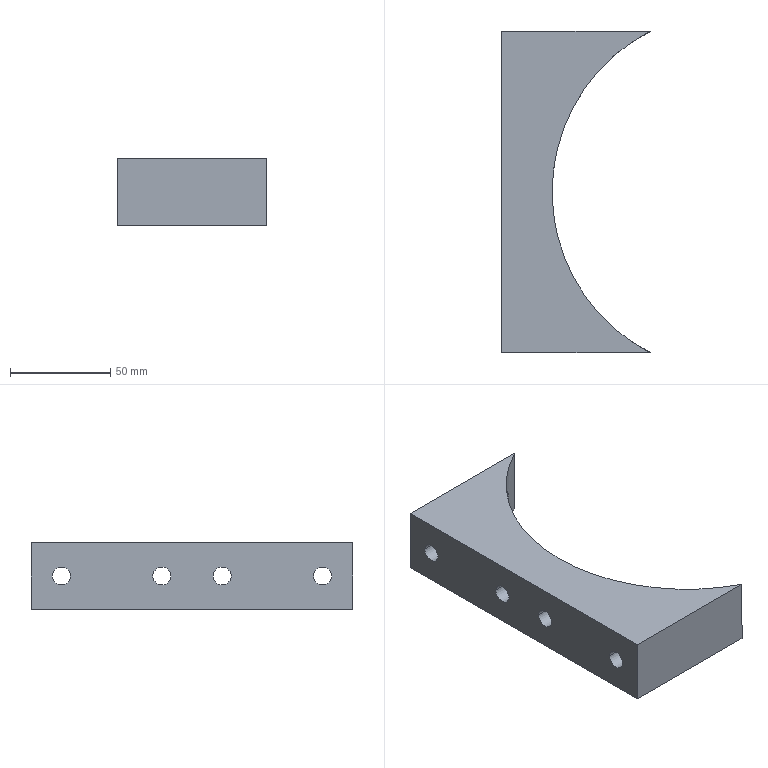Component | SolidWorks | ClampingAssembly-2_BrakeBlock-1 | 1 solid | 26 faces | box 73.77 x 160 x 33 mm | volume 180538 mm3 | cylinder 17 | plane 9 | commonest cylinder face diameters 15 x8 9 x8 180 x1 | material Industrial Rubber Sheet
build123d program:
from build123d import *

# Parameters (mm, degrees)
SKETCH1_W                                       = 160
SKETCH1_H                                       = 33
BOSS_EXTRUDE1_DEPTH                             = 75
M8_HEX_SOCKET_HEAD_CAP_SCREW_CBORE1_D           = 9
M8_HEX_SOCKET_HEAD_CAP_SCREW_CBORE1_CBORE_D     = 15
M8_HEX_SOCKET_HEAD_CAP_SCREW_CBORE1_CBORE_DEPTH = 68.6
SKETCH4_R                                       = 90
CUT_EXTRUDE1_DEPTH                              = 115.516


with BuildPart() as part:
    # Sketch1 → Boss-Extrude1 (new body)
    with BuildSketch(Plane.XY):
        Rectangle(SKETCH1_W, SKETCH1_H)
    extrude(amount=BOSS_EXTRUDE1_DEPTH)

    # M8 Hex Socket Head Cap Screw CBORE1 (through all)
    with Locations(Plane(origin=(-65, 0, 75), x_dir=(1, 0, 0), z_dir=(0, 0, 1))):
        with Locations((0, 0), (50, 0), (80, 0), (130, 0)):
            CounterBoreHole(M8_HEX_SOCKET_HEAD_CAP_SCREW_CBORE1_D / 2, M8_HEX_SOCKET_HEAD_CAP_SCREW_CBORE1_CBORE_D / 2, M8_HEX_SOCKET_HEAD_CAP_SCREW_CBORE1_CBORE_DEPTH)

    # Sketch4 → Cut-Extrude1 (cut, through all)
    with BuildSketch(Plane(origin=(0, 16.5, 0), x_dir=(1, 0, 0), z_dir=(0, 1, 0))):
        with Locations((0, -115)):
            Circle(SKETCH4_R)
    extrude(amount=-CUT_EXTRUDE1_DEPTH, mode=Mode.SUBTRACT)


solid = part.part

# Placed as in the assembly
solid = solid.moved(Location((-116.365, -26.917, -1210.457), (90, 90, 0)))